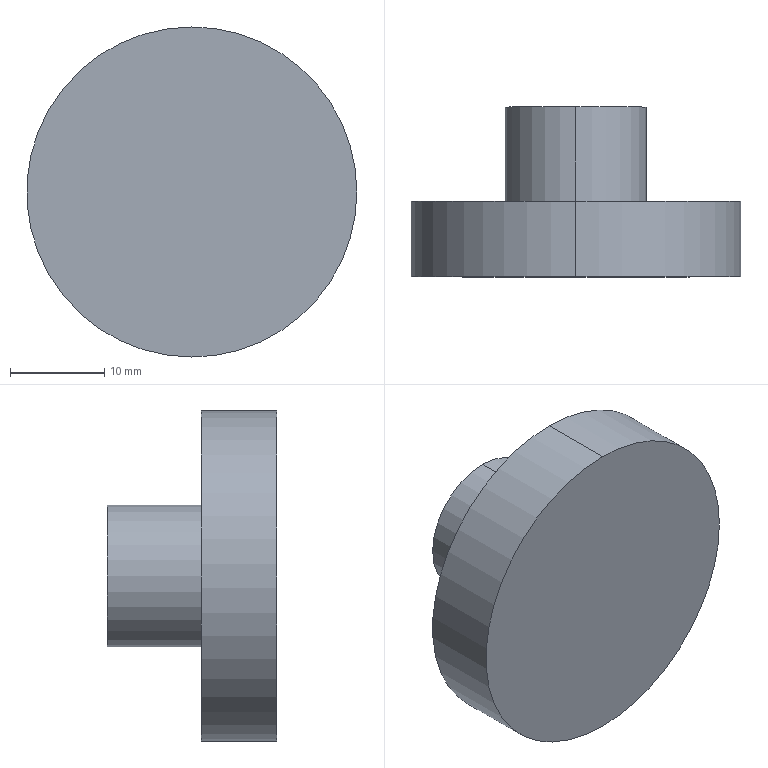CAM job | Mastercam | mm | 1 operations | part box 35 x 18 x 35
1. Drill/Counterbore | 7 - 4 倒角刀